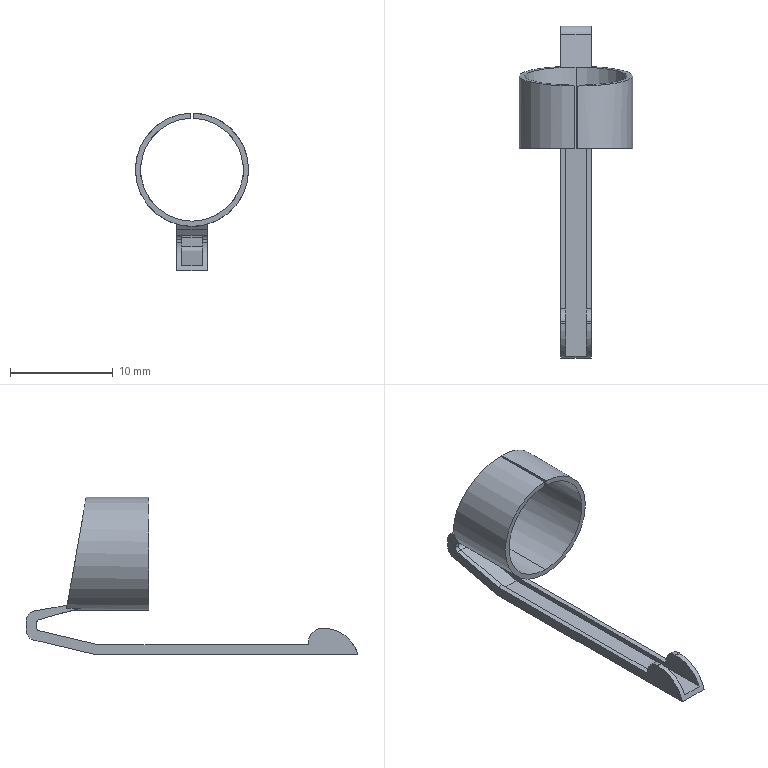Component | SolidWorks | PenHolder-1 | 1 solid | 43 faces | volume 196 mm3 | plane 26 | cylinder 17 | commonest cylinder face diameters 0.8 x4 7.021 x3 10 x2 11 x2 2.732 x2 2 x2 1 x2